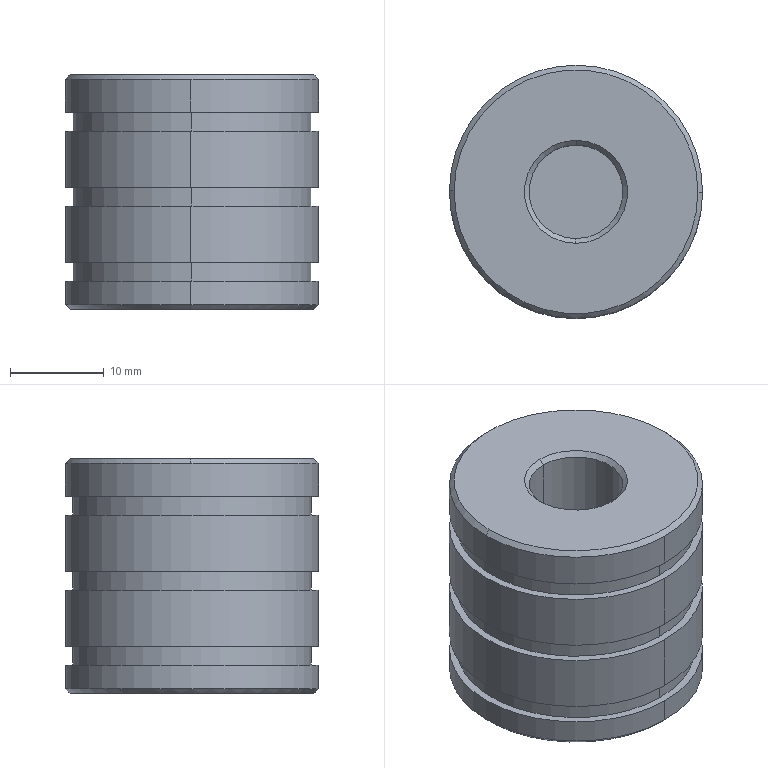Component | SolidWorks | YC1-250-09SecondDropAssembly-1_Coupling-1 | 1 solid | 36 faces | box 27 x 27 x 25 mm | volume 12319 mm3 | cylinder 18 | plane 10 | cone 8 | commonest cylinder face diameters 27 x8 25.4 x6 10 x4 | material Plain Carbon Steel
STEP:
#1=CARTESIAN_POINT('',(0.004281,132.205,-42.775));
#2=VERTEX_POINT('',#1);
#3=CARTESIAN_POINT('',(-0.004281,131.181,-42.775));
#4=VERTEX_POINT('',#3);
#5=CARTESIAN_POINT('',(0.,131.693,-42.775));
#6=DIRECTION('',(0.,0.,1.));
#7=DIRECTION('',(0.008365,1.,0.));
#8=AXIS2_PLACEMENT_3D('',#5,#6,#7);
#9=CIRCLE('',#8,0.5118);
#10=EDGE_CURVE('',#2,#4,#9,.T.);
#11=ORIENTED_EDGE('',*,*,#10,.T.);
#12=CARTESIAN_POINT('',(-0.004446,131.161,-42.755));
#13=VERTEX_POINT('',#12);
#14=CARTESIAN_POINT('',(-0.004446,131.161,-42.755));
#15=DIRECTION('',(-0.005915,-0.7071,0.7071));
#16=VECTOR('',#15,39.37);
#17=LINE('',#14,#16);
#18=EDGE_CURVE('',#4,#13,#17,.T.);
#19=ORIENTED_EDGE('',*,*,#18,.T.);
#20=CARTESIAN_POINT('',(0.004446,132.224,-42.755));
#21=VERTEX_POINT('',#20);
#22=CARTESIAN_POINT('',(0.,131.693,-42.755));
#23=DIRECTION('',(0.,0.,-1.));
#24=DIRECTION('',(0.008365,1.,0.));
#25=AXIS2_PLACEMENT_3D('',#22,#23,#24);
#26=CIRCLE('',#25,0.5315);
#27=EDGE_CURVE('',#13,#21,#26,.T.);
#28=ORIENTED_EDGE('',*,*,#27,.T.);
#29=CARTESIAN_POINT('',(0.004446,132.224,-42.755));
#30=DIRECTION('',(0.005915,0.7071,0.7071));
#31=VECTOR('',#30,39.37);
#32=LINE('',#29,#31);
#33=EDGE_CURVE('',#2,#21,#32,.T.);
#34=ORIENTED_EDGE('',*,*,#33,.F.);
#35=EDGE_LOOP('',(#11,#19,#28,#34));
#36=FACE_OUTER_BOUND('',#35,.T.);
#37=CARTESIAN_POINT('',(0.,131.693,-42.755));
#38=DIRECTION('',(0.,0.,1.));
#39=DIRECTION('',(0.008365,1.,0.));
#40=AXIS2_PLACEMENT_3D('',#37,#38,#39);
#41=CONICAL_SURFACE('',#40,0.5315,0.7854);
#42=ADVANCED_FACE('',(#36),#41,.T.);
#43=CARTESIAN_POINT('',(0.1968,131.691,-42.755));
#44=VERTEX_POINT('',#43);
#45=CARTESIAN_POINT('',(-0.001647,131.496,-42.755));
#46=VERTEX_POINT('',#45);
#47=CARTESIAN_POINT('',(0.,131.693,-42.755));
#48=DIRECTION('',(0.,0.,-1.));
#49=DIRECTION('',(-0.008365,-1.,0.));
#50=AXIS2_PLACEMENT_3D('',#47,#48,#49);
#51=CIRCLE('',#50,0.1969);
#52=EDGE_CURVE('',#44,#46,#51,.T.);
#53=ORIENTED_EDGE('',*,*,#52,.F.);
#54=CARTESIAN_POINT('',(0.2165,131.691,-42.775));
#55=VERTEX_POINT('',#54);
#56=CARTESIAN_POINT('',(0.2165,131.691,-42.775));
#57=DIRECTION('',(0.7071,-0.005915,-0.7071));
#58=VECTOR('',#57,39.37);
#59=LINE('',#56,#58);
#60=EDGE_CURVE('',#44,#55,#59,.T.);
#61=ORIENTED_EDGE('',*,*,#60,.T.);
#62=CARTESIAN_POINT('',(-0.2165,131.695,-42.775));
#63=VERTEX_POINT('',#62);
#64=CARTESIAN_POINT('',(0.,131.693,-42.775));
#65=DIRECTION('',(-0.,0.,-1.));
#66=DIRECTION('',(-1.,0.008365,0.));
#67=AXIS2_PLACEMENT_3D('',#64,#65,#66);
#68=CIRCLE('',#67,0.2165);
#69=EDGE_CURVE('',#55,#63,#68,.T.);
#70=ORIENTED_EDGE('',*,*,#69,.T.);
#71=CARTESIAN_POINT('',(-0.1968,131.695,-42.755));
#72=VERTEX_POINT('',#71);
#73=CARTESIAN_POINT('',(-0.2165,131.695,-42.775));
#74=DIRECTION('',(-0.7071,0.005915,-0.7071));
#75=VECTOR('',#74,39.37);
#76=LINE('',#73,#75);
#77=EDGE_CURVE('',#72,#63,#76,.T.);
#78=ORIENTED_EDGE('',*,*,#77,.F.);
#79=CARTESIAN_POINT('',(0.,131.693,-42.755));
#80=DIRECTION('',(0.,0.,-1.));
#81=DIRECTION('',(-0.008365,-1.,0.));
#82=AXIS2_PLACEMENT_3D('',#79,#80,#81);
#83=CIRCLE('',#82,0.1969);
#84=EDGE_CURVE('',#46,#72,#83,.T.);
#85=ORIENTED_EDGE('',*,*,#84,.F.);
#86=EDGE_LOOP('',(#53,#61,#70,#78,#85));
#87=FACE_OUTER_BOUND('',#86,.T.);
#88=CARTESIAN_POINT('',(0.,131.693,-42.775));
#89=DIRECTION('',(-0.,0.,-1.));
#90=DIRECTION('',(-1.,0.008365,0.));
#91=AXIS2_PLACEMENT_3D('',#88,#89,#90);
#92=CONICAL_SURFACE('',#91,0.2165,0.7854);
#93=ADVANCED_FACE('',(#87),#92,.F.);
#94=ORIENTED_EDGE('',*,*,#27,.F.);
#95=CARTESIAN_POINT('',(-0.004446,131.161,-42.657));
#96=VERTEX_POINT('',#95);
#97=CARTESIAN_POINT('',(-0.004446,131.161,-41.79));
#98=DIRECTION('',(0.,0.,1.));
#99=VECTOR('',#98,39.37);
#100=LINE('',#97,#99);
#101=EDGE_CURVE('',#13,#96,#100,.T.);
#102=ORIENTED_EDGE('',*,*,#101,.T.);
#103=CARTESIAN_POINT('',(0.004446,132.224,-42.657));
#104=VERTEX_POINT('',#103);
#105=CARTESIAN_POINT('',(0.,131.693,-42.657));
#106=DIRECTION('',(0.,0.,-1.));
#107=DIRECTION('',(0.008365,1.,0.));
#108=AXIS2_PLACEMENT_3D('',#105,#106,#107);
#109=CIRCLE('',#108,0.5315);
#110=EDGE_CURVE('',#96,#104,#109,.T.);
#111=ORIENTED_EDGE('',*,*,#110,.T.);
#112=CARTESIAN_POINT('',(0.004446,132.224,-41.79));
#113=DIRECTION('',(0.,0.,1.));
#114=VECTOR('',#113,39.37);
#115=LINE('',#112,#114);
#116=EDGE_CURVE('',#21,#104,#115,.T.);
#117=ORIENTED_EDGE('',*,*,#116,.F.);
#118=EDGE_LOOP('',(#94,#102,#111,#117));
#119=FACE_OUTER_BOUND('',#118,.T.);
#120=CARTESIAN_POINT('',(0.,131.693,-41.79));
#121=DIRECTION('',(0.,0.,1.));
#122=DIRECTION('',(0.008365,1.,0.));
#123=AXIS2_PLACEMENT_3D('',#120,#121,#122);
#124=CYLINDRICAL_SURFACE('',#123,0.5315);
#125=ADVANCED_FACE('',(#119),#124,.T.);
#126=CARTESIAN_POINT('',(0.001647,131.89,-42.755));
#127=VERTEX_POINT('',#126);
#128=CARTESIAN_POINT('',(0.,131.693,-42.755));
#129=DIRECTION('',(0.,0.,-1.));
#130=DIRECTION('',(-0.008365,-1.,0.));
#131=AXIS2_PLACEMENT_3D('',#128,#129,#130);
#132=CIRCLE('',#131,0.1969);
#133=EDGE_CURVE('',#127,#44,#132,.T.);
#134=ORIENTED_EDGE('',*,*,#133,.T.);
#135=ORIENTED_EDGE('',*,*,#52,.T.);
#136=CARTESIAN_POINT('',(-0.001647,131.496,-42.381));
#137=VERTEX_POINT('',#136);
#138=CARTESIAN_POINT('',(-0.001647,131.496,-41.79));
#139=DIRECTION('',(0.,0.,1.));
#140=VECTOR('',#139,39.37);
#141=LINE('',#138,#140);
#142=EDGE_CURVE('',#46,#137,#141,.T.);
#143=ORIENTED_EDGE('',*,*,#142,.T.);
#144=CARTESIAN_POINT('',(0.001647,131.89,-42.381));
#145=VERTEX_POINT('',#144);
#146=CARTESIAN_POINT('',(0.,131.693,-42.381));
#147=DIRECTION('',(0.,0.,-1.));
#148=DIRECTION('',(0.008365,1.,0.));
#149=AXIS2_PLACEMENT_3D('',#146,#147,#148);
#150=CIRCLE('',#149,0.1969);
#151=EDGE_CURVE('',#145,#137,#150,.T.);
#152=ORIENTED_EDGE('',*,*,#151,.F.);
#153=CARTESIAN_POINT('',(0.001647,131.89,-41.79));
#154=DIRECTION('',(0.,0.,1.));
#155=VECTOR('',#154,39.37);
#156=LINE('',#153,#155);
#157=EDGE_CURVE('',#127,#145,#156,.T.);
#158=ORIENTED_EDGE('',*,*,#157,.F.);
#159=EDGE_LOOP('',(#134,#135,#143,#152,#158));
#160=FACE_OUTER_BOUND('',#159,.T.);
#161=CARTESIAN_POINT('',(0.,131.693,-41.79));
#162=DIRECTION('',(0.,0.,1.));
#163=DIRECTION('',(0.008365,1.,0.));
#164=AXIS2_PLACEMENT_3D('',#161,#162,#163);
#165=CYLINDRICAL_SURFACE('',#164,0.1969);
#166=ADVANCED_FACE('',(#160),#165,.F.);
#167=CARTESIAN_POINT('',(-0.004183,131.193,-42.578));
#168=VERTEX_POINT('',#167);
#169=CARTESIAN_POINT('',(0.004183,132.193,-42.578));
#170=VERTEX_POINT('',#169);
#171=CARTESIAN_POINT('',(0.,131.693,-42.578));
#172=DIRECTION('',(0.,0.,-1.));
#173=DIRECTION('',(-0.008365,-1.,0.));
#174=AXIS2_PLACEMENT_3D('',#171,#172,#173);
#175=CIRCLE('',#174,0.5);
#176=EDGE_CURVE('',#168,#170,#175,.T.);
#177=ORIENTED_EDGE('',*,*,#176,.T.);
#178=CARTESIAN_POINT('',(0.004183,132.193,-42.657));
#179=VERTEX_POINT('',#178);
#180=CARTESIAN_POINT('',(0.004183,132.193,-42.578));
#181=DIRECTION('',(0.,0.,-1.));
#182=VECTOR('',#181,39.37);
#183=LINE('',#180,#182);
#184=EDGE_CURVE('',#170,#179,#183,.T.);
#185=ORIENTED_EDGE('',*,*,#184,.T.);
#186=CARTESIAN_POINT('',(-0.004183,131.193,-42.657));
#187=VERTEX_POINT('',#186);
#188=CARTESIAN_POINT('',(0.,131.693,-42.657));
#189=DIRECTION('',(0.,0.,1.));
#190=DIRECTION('',(-0.008365,-1.,0.));
#191=AXIS2_PLACEMENT_3D('',#188,#189,#190);
#192=CIRCLE('',#191,0.5);
#193=EDGE_CURVE('',#179,#187,#192,.T.);
#194=ORIENTED_EDGE('',*,*,#193,.T.);
#195=CARTESIAN_POINT('',(-0.004183,131.193,-42.578));
#196=DIRECTION('',(0.,0.,-1.));
#197=VECTOR('',#196,39.37);
#198=LINE('',#195,#197);
#199=EDGE_CURVE('',#168,#187,#198,.T.);
#200=ORIENTED_EDGE('',*,*,#199,.F.);
#201=EDGE_LOOP('',(#177,#185,#194,#200));
#202=FACE_OUTER_BOUND('',#201,.T.);
#203=CARTESIAN_POINT('',(0.,131.693,-42.578));
#204=DIRECTION('',(0.,0.,-1.));
#205=DIRECTION('',(-0.008365,-1.,0.));
#206=AXIS2_PLACEMENT_3D('',#203,#204,#205);
#207=CYLINDRICAL_SURFACE('',#206,0.5);
#208=ADVANCED_FACE('',(#202),#207,.T.);
#209=CARTESIAN_POINT('',(0.004446,132.224,-42.578));
#210=VERTEX_POINT('',#209);
#211=CARTESIAN_POINT('',(-0.004446,131.161,-42.578));
#212=VERTEX_POINT('',#211);
#213=CARTESIAN_POINT('',(0.,131.693,-42.578));
#214=DIRECTION('',(0.,0.,1.));
#215=DIRECTION('',(0.008365,1.,0.));
#216=AXIS2_PLACEMENT_3D('',#213,#214,#215);
#217=CIRCLE('',#216,0.5315);
#218=EDGE_CURVE('',#210,#212,#217,.T.);
#219=ORIENTED_EDGE('',*,*,#218,.T.);
#220=CARTESIAN_POINT('',(-0.004446,131.161,-42.342));
#221=VERTEX_POINT('',#220);
#222=CARTESIAN_POINT('',(-0.004446,131.161,-41.79));
#223=DIRECTION('',(0.,0.,1.));
#224=VECTOR('',#223,39.37);
#225=LINE('',#222,#224);
#226=EDGE_CURVE('',#212,#221,#225,.T.);
#227=ORIENTED_EDGE('',*,*,#226,.T.);
#228=CARTESIAN_POINT('',(0.004446,132.224,-42.342));
#229=VERTEX_POINT('',#228);
#230=CARTESIAN_POINT('',(0.,131.693,-42.342));
#231=DIRECTION('',(0.,0.,-1.));
#232=DIRECTION('',(0.008365,1.,0.));
#233=AXIS2_PLACEMENT_3D('',#230,#231,#232);
#234=CIRCLE('',#233,0.5315);
#235=EDGE_CURVE('',#221,#229,#234,.T.);
#236=ORIENTED_EDGE('',*,*,#235,.T.);
#237=CARTESIAN_POINT('',(0.004446,132.224,-41.79));
#238=DIRECTION('',(0.,0.,1.));
#239=VECTOR('',#238,39.37);
#240=LINE('',#237,#239);
#241=EDGE_CURVE('',#210,#229,#240,.T.);
#242=ORIENTED_EDGE('',*,*,#241,.F.);
#243=EDGE_LOOP('',(#219,#227,#236,#242));
#244=FACE_OUTER_BOUND('',#243,.T.);
#245=CARTESIAN_POINT('',(0.,131.693,-41.79));
#246=DIRECTION('',(0.,0.,1.));
#247=DIRECTION('',(0.008365,1.,0.));
#248=AXIS2_PLACEMENT_3D('',#245,#246,#247);
#249=CYLINDRICAL_SURFACE('',#248,0.5315);
#250=ADVANCED_FACE('',(#244),#249,.T.);
#251=CARTESIAN_POINT('',(-0.004183,131.193,-42.263));
#252=VERTEX_POINT('',#251);
#253=CARTESIAN_POINT('',(0.004183,132.193,-42.263));
#254=VERTEX_POINT('',#253);
#255=CARTESIAN_POINT('',(0.,131.693,-42.263));
#256=DIRECTION('',(0.,0.,-1.));
#257=DIRECTION('',(-0.008365,-1.,0.));
#258=AXIS2_PLACEMENT_3D('',#255,#256,#257);
#259=CIRCLE('',#258,0.5);
#260=EDGE_CURVE('',#252,#254,#259,.T.);
#261=ORIENTED_EDGE('',*,*,#260,.T.);
#262=CARTESIAN_POINT('',(0.004183,132.193,-42.342));
#263=VERTEX_POINT('',#262);
#264=CARTESIAN_POINT('',(0.004183,132.193,-42.263));
#265=DIRECTION('',(0.,0.,-1.));
#266=VECTOR('',#265,39.37);
#267=LINE('',#264,#266);
#268=EDGE_CURVE('',#254,#263,#267,.T.);
#269=ORIENTED_EDGE('',*,*,#268,.T.);
#270=CARTESIAN_POINT('',(-0.004183,131.193,-42.342));
#271=VERTEX_POINT('',#270);
#272=CARTESIAN_POINT('',(0.,131.693,-42.342));
#273=DIRECTION('',(0.,0.,1.));
#274=DIRECTION('',(-0.008365,-1.,0.));
#275=AXIS2_PLACEMENT_3D('',#272,#273,#274);
#276=CIRCLE('',#275,0.5);
#277=EDGE_CURVE('',#263,#271,#276,.T.);
#278=ORIENTED_EDGE('',*,*,#277,.T.);
#279=CARTESIAN_POINT('',(-0.004183,131.193,-42.263));
#280=DIRECTION('',(0.,0.,-1.));
#281=VECTOR('',#280,39.37);
#282=LINE('',#279,#281);
#283=EDGE_CURVE('',#252,#271,#282,.T.);
#284=ORIENTED_EDGE('',*,*,#283,.F.);
#285=EDGE_LOOP('',(#261,#269,#278,#284));
#286=FACE_OUTER_BOUND('',#285,.T.);
#287=CARTESIAN_POINT('',(0.,131.693,-42.263));
#288=DIRECTION('',(0.,0.,-1.));
#289=DIRECTION('',(-0.008365,-1.,0.));
#290=AXIS2_PLACEMENT_3D('',#287,#288,#289);
#291=CYLINDRICAL_SURFACE('',#290,0.5);
#292=ADVANCED_FACE('',(#286),#291,.T.);
#293=CARTESIAN_POINT('',(0.004446,132.224,-42.263));
#294=VERTEX_POINT('',#293);
#295=CARTESIAN_POINT('',(-0.004446,131.161,-42.263));
#296=VERTEX_POINT('',#295);
#297=CARTESIAN_POINT('',(0.,131.693,-42.263));
#298=DIRECTION('',(0.,0.,1.));
#299=DIRECTION('',(0.008365,1.,0.));
#300=AXIS2_PLACEMENT_3D('',#297,#298,#299);
#301=CIRCLE('',#300,0.5315);
#302=EDGE_CURVE('',#294,#296,#301,.T.);
#303=ORIENTED_EDGE('',*,*,#302,.T.);
#304=CARTESIAN_POINT('',(-0.004446,131.161,-42.027));
#305=VERTEX_POINT('',#304);
#306=CARTESIAN_POINT('',(-0.004446,131.161,-41.79));
#307=DIRECTION('',(0.,0.,1.));
#308=VECTOR('',#307,39.37);
#309=LINE('',#306,#308);
#310=EDGE_CURVE('',#296,#305,#309,.T.);
#311=ORIENTED_EDGE('',*,*,#310,.T.);
#312=CARTESIAN_POINT('',(0.004446,132.224,-42.027));
#313=VERTEX_POINT('',#312);
#314=CARTESIAN_POINT('',(0.,131.693,-42.027));
#315=DIRECTION('',(0.,0.,-1.));
#316=DIRECTION('',(0.008365,1.,0.));
#317=AXIS2_PLACEMENT_3D('',#314,#315,#316);
#318=CIRCLE('',#317,0.5315);
#319=EDGE_CURVE('',#305,#313,#318,.T.);
#320=ORIENTED_EDGE('',*,*,#319,.T.);
#321=CARTESIAN_POINT('',(0.004446,132.224,-41.79));
#322=DIRECTION('',(0.,0.,1.));
#323=VECTOR('',#322,39.37);
#324=LINE('',#321,#323);
#325=EDGE_CURVE('',#294,#313,#324,.T.);
#326=ORIENTED_EDGE('',*,*,#325,.F.);
#327=EDGE_LOOP('',(#303,#311,#320,#326));
#328=FACE_OUTER_BOUND('',#327,.T.);
#329=CARTESIAN_POINT('',(0.,131.693,-41.79));
#330=DIRECTION('',(0.,0.,1.));
#331=DIRECTION('',(0.008365,1.,0.));
#332=AXIS2_PLACEMENT_3D('',#329,#330,#331);
#333=CYLINDRICAL_SURFACE('',#332,0.5315);
#334=ADVANCED_FACE('',(#328),#333,.T.);
#335=CARTESIAN_POINT('',(-0.004183,131.193,-41.948));
#336=VERTEX_POINT('',#335);
#337=CARTESIAN_POINT('',(0.004183,132.193,-41.948));
#338=VERTEX_POINT('',#337);
#339=CARTESIAN_POINT('',(0.,131.693,-41.948));
#340=DIRECTION('',(0.,0.,-1.));
#341=DIRECTION('',(-0.008365,-1.,0.));
#342=AXIS2_PLACEMENT_3D('',#339,#340,#341);
#343=CIRCLE('',#342,0.5);
#344=EDGE_CURVE('',#336,#338,#343,.T.);
#345=ORIENTED_EDGE('',*,*,#344,.T.);
#346=CARTESIAN_POINT('',(0.004183,132.193,-42.027));
#347=VERTEX_POINT('',#346);
#348=CARTESIAN_POINT('',(0.004183,132.193,-42.755));
#349=DIRECTION('',(0.,0.,-1.));
#350=VECTOR('',#349,39.37);
#351=LINE('',#348,#350);
#352=EDGE_CURVE('',#338,#347,#351,.T.);
#353=ORIENTED_EDGE('',*,*,#352,.T.);
#354=CARTESIAN_POINT('',(-0.004183,131.193,-42.027));
#355=VERTEX_POINT('',#354);
#356=CARTESIAN_POINT('',(0.,131.693,-42.027));
#357=DIRECTION('',(0.,0.,1.));
#358=DIRECTION('',(-0.008365,-1.,0.));
#359=AXIS2_PLACEMENT_3D('',#356,#357,#358);
#360=CIRCLE('',#359,0.5);
#361=EDGE_CURVE('',#347,#355,#360,.T.);
#362=ORIENTED_EDGE('',*,*,#361,.T.);
#363=CARTESIAN_POINT('',(-0.004183,131.193,-42.755));
#364=DIRECTION('',(0.,0.,-1.));
#365=VECTOR('',#364,39.37);
#366=LINE('',#363,#365);
#367=EDGE_CURVE('',#336,#355,#366,.T.);
#368=ORIENTED_EDGE('',*,*,#367,.F.);
#369=EDGE_LOOP('',(#345,#353,#362,#368));
#370=FACE_OUTER_BOUND('',#369,.T.);
#371=CARTESIAN_POINT('',(0.,131.693,-42.755));
#372=DIRECTION('',(0.,0.,-1.));
#373=DIRECTION('',(-0.008365,-1.,0.));
#374=AXIS2_PLACEMENT_3D('',#371,#372,#373);
#375=CYLINDRICAL_SURFACE('',#374,0.5);
#376=ADVANCED_FACE('',(#370),#375,.T.);
#377=CARTESIAN_POINT('',(0.004446,132.224,-41.948));
#378=VERTEX_POINT('',#377);
#379=CARTESIAN_POINT('',(-0.004446,131.161,-41.948));
#380=VERTEX_POINT('',#379);
#381=CARTESIAN_POINT('',(0.,131.693,-41.948));
#382=DIRECTION('',(0.,0.,1.));
#383=DIRECTION('',(0.008365,1.,0.));
#384=AXIS2_PLACEMENT_3D('',#381,#382,#383);
#385=CIRCLE('',#384,0.5315);
#386=EDGE_CURVE('',#378,#380,#385,.T.);
#387=ORIENTED_EDGE('',*,*,#386,.T.);
#388=CARTESIAN_POINT('',(-0.004446,131.161,-41.81));
#389=VERTEX_POINT('',#388);
#390=CARTESIAN_POINT('',(-0.004446,131.161,-41.79));
#391=DIRECTION('',(0.,0.,1.));
#392=VECTOR('',#391,39.37);
#393=LINE('',#390,#392);
#394=EDGE_CURVE('',#380,#389,#393,.T.);
#395=ORIENTED_EDGE('',*,*,#394,.T.);
#396=CARTESIAN_POINT('',(-0.5315,131.697,-41.81));
#397=VERTEX_POINT('',#396);
#398=CARTESIAN_POINT('',(0.,131.693,-41.81));
#399=DIRECTION('',(0.,0.,-1.));
#400=DIRECTION('',(0.008365,1.,0.));
#401=AXIS2_PLACEMENT_3D('',#398,#399,#400);
#402=CIRCLE('',#401,0.5315);
#403=EDGE_CURVE('',#389,#397,#402,.T.);
#404=ORIENTED_EDGE('',*,*,#403,.T.);
#405=CARTESIAN_POINT('',(0.004446,132.224,-41.81));
#406=VERTEX_POINT('',#405);
#407=CARTESIAN_POINT('',(0.,131.693,-41.81));
#408=DIRECTION('',(0.,0.,-1.));
#409=DIRECTION('',(0.008365,1.,0.));
#410=AXIS2_PLACEMENT_3D('',#407,#408,#409);
#411=CIRCLE('',#410,0.5315);
#412=EDGE_CURVE('',#397,#406,#411,.T.);
#413=ORIENTED_EDGE('',*,*,#412,.T.);
#414=CARTESIAN_POINT('',(0.004446,132.224,-41.79));
#415=DIRECTION('',(0.,0.,1.));
#416=VECTOR('',#415,39.37);
#417=LINE('',#414,#416);
#418=EDGE_CURVE('',#378,#406,#417,.T.);
#419=ORIENTED_EDGE('',*,*,#418,.F.);
#420=EDGE_LOOP('',(#387,#395,#404,#413,#419));
#421=FACE_OUTER_BOUND('',#420,.T.);
#422=CARTESIAN_POINT('',(0.,131.693,-41.79));
#423=DIRECTION('',(0.,0.,1.));
#424=DIRECTION('',(0.008365,1.,0.));
#425=AXIS2_PLACEMENT_3D('',#422,#423,#424);
#426=CYLINDRICAL_SURFACE('',#425,0.5315);
#427=ADVANCED_FACE('',(#421),#426,.T.);
#428=CARTESIAN_POINT('',(-0.5118,131.697,-41.79));
#429=VERTEX_POINT('',#428);
#430=CARTESIAN_POINT('',(0.5118,131.689,-41.79));
#431=VERTEX_POINT('',#430);
#432=CARTESIAN_POINT('',(0.,131.693,-41.79));
#433=DIRECTION('',(-0.,0.,-1.));
#434=DIRECTION('',(-1.,0.008365,0.));
#435=AXIS2_PLACEMENT_3D('',#432,#433,#434);
#436=CIRCLE('',#435,0.5118);
#437=EDGE_CURVE('',#429,#431,#436,.T.);
#438=ORIENTED_EDGE('',*,*,#437,.T.);
#439=CARTESIAN_POINT('',(0.5315,131.688,-41.81));
#440=VERTEX_POINT('',#439);
#441=CARTESIAN_POINT('',(0.5315,131.688,-41.81));
#442=DIRECTION('',(0.7071,-0.005915,-0.7071));
#443=VECTOR('',#442,39.37);
#444=LINE('',#441,#443);
#445=EDGE_CURVE('',#431,#440,#444,.T.);
#446=ORIENTED_EDGE('',*,*,#445,.T.);
#447=CARTESIAN_POINT('',(0.,131.693,-41.81));
#448=DIRECTION('',(0.,0.,-1.));
#449=DIRECTION('',(0.008365,1.,0.));
#450=AXIS2_PLACEMENT_3D('',#447,#448,#449);
#451=CIRCLE('',#450,0.5315);
#452=EDGE_CURVE('',#406,#440,#451,.T.);
#453=ORIENTED_EDGE('',*,*,#452,.F.);
#454=ORIENTED_EDGE('',*,*,#412,.F.);
#455=CARTESIAN_POINT('',(-0.5315,131.697,-41.81));
#456=DIRECTION('',(-0.7071,0.005915,-0.7071));
#457=VECTOR('',#456,39.37);
#458=LINE('',#455,#457);
#459=EDGE_CURVE('',#429,#397,#458,.T.);
#460=ORIENTED_EDGE('',*,*,#459,.F.);
#461=EDGE_LOOP('',(#438,#446,#453,#454,#460));
#462=FACE_OUTER_BOUND('',#461,.T.);
#463=CARTESIAN_POINT('',(0.,131.693,-41.81));
#464=DIRECTION('',(-0.,0.,-1.));
#465=DIRECTION('',(-1.,0.008365,0.));
#466=AXIS2_PLACEMENT_3D('',#463,#464,#465);
#467=CONICAL_SURFACE('',#466,0.5315,0.7854);
#468=ADVANCED_FACE('',(#462),#467,.T.);
#469=CARTESIAN_POINT('',(-0.001647,131.496,-41.81));
#470=VERTEX_POINT('',#469);
#471=CARTESIAN_POINT('',(0.001647,131.89,-41.81));
#472=VERTEX_POINT('',#471);
#473=CARTESIAN_POINT('',(0.,131.693,-41.81));
#474=DIRECTION('',(0.,0.,1.));
#475=DIRECTION('',(0.008365,1.,0.));
#476=AXIS2_PLACEMENT_3D('',#473,#474,#475);
#477=CIRCLE('',#476,0.1969);
#478=EDGE_CURVE('',#470,#472,#477,.T.);
#479=ORIENTED_EDGE('',*,*,#478,.F.);
#480=CARTESIAN_POINT('',(-0.001811,131.476,-41.79));
#481=VERTEX_POINT('',#480);
#482=CARTESIAN_POINT('',(-0.001811,131.476,-41.79));
#483=DIRECTION('',(-0.005915,-0.7071,0.7071));
#484=VECTOR('',#483,39.37);
#485=LINE('',#482,#484);
#486=EDGE_CURVE('',#470,#481,#485,.T.);
#487=ORIENTED_EDGE('',*,*,#486,.T.);
#488=CARTESIAN_POINT('',(0.001811,131.909,-41.79));
#489=VERTEX_POINT('',#488);
#490=CARTESIAN_POINT('',(0.,131.693,-41.79));
#491=DIRECTION('',(0.,0.,1.));
#492=DIRECTION('',(0.008365,1.,0.));
#493=AXIS2_PLACEMENT_3D('',#490,#491,#492);
#494=CIRCLE('',#493,0.2165);
#495=EDGE_CURVE('',#481,#489,#494,.T.);
#496=ORIENTED_EDGE('',*,*,#495,.T.);
#497=CARTESIAN_POINT('',(0.001811,131.909,-41.79));
#498=DIRECTION('',(0.005915,0.7071,0.7071));
#499=VECTOR('',#498,39.37);
#500=LINE('',#497,#499);
#501=EDGE_CURVE('',#472,#489,#500,.T.);
#502=ORIENTED_EDGE('',*,*,#501,.F.);
#503=EDGE_LOOP('',(#479,#487,#496,#502));
#504=FACE_OUTER_BOUND('',#503,.T.);
#505=CARTESIAN_POINT('',(0.,131.693,-41.79));
#506=DIRECTION('',(0.,0.,1.));
#507=DIRECTION('',(0.008365,1.,0.));
#508=AXIS2_PLACEMENT_3D('',#505,#506,#507);
#509=CONICAL_SURFACE('',#508,0.2165,0.7854);
#510=ADVANCED_FACE('',(#504),#509,.F.);
#511=CARTESIAN_POINT('',(-0.001647,131.496,-42.184));
#512=VERTEX_POINT('',#511);
#513=CARTESIAN_POINT('',(0.001647,131.89,-42.184));
#514=VERTEX_POINT('',#513);
#515=CARTESIAN_POINT('',(0.,131.693,-42.184));
#516=DIRECTION('',(0.,0.,1.));
#517=DIRECTION('',(0.008365,1.,0.));
#518=AXIS2_PLACEMENT_3D('',#515,#516,#517);
#519=CIRCLE('',#518,0.1969);
#520=EDGE_CURVE('',#512,#514,#519,.T.);
#521=ORIENTED_EDGE('',*,*,#520,.F.);
#522=CARTESIAN_POINT('',(-0.001647,131.496,-41.79));
#523=DIRECTION('',(0.,0.,1.));
#524=VECTOR('',#523,39.37);
#525=LINE('',#522,#524);
#526=EDGE_CURVE('',#512,#470,#525,.T.);
#527=ORIENTED_EDGE('',*,*,#526,.T.);
#528=ORIENTED_EDGE('',*,*,#478,.T.);
#529=CARTESIAN_POINT('',(0.001647,131.89,-41.79));
#530=DIRECTION('',(0.,0.,1.));
#531=VECTOR('',#530,39.37);
#532=LINE('',#529,#531);
#533=EDGE_CURVE('',#514,#472,#532,.T.);
#534=ORIENTED_EDGE('',*,*,#533,.F.);
#535=EDGE_LOOP('',(#521,#527,#528,#534));
#536=FACE_OUTER_BOUND('',#535,.T.);
#537=CARTESIAN_POINT('',(0.,131.693,-41.79));
#538=DIRECTION('',(0.,0.,1.));
#539=DIRECTION('',(0.008365,1.,0.));
#540=AXIS2_PLACEMENT_3D('',#537,#538,#539);
#541=CYLINDRICAL_SURFACE('',#540,0.1969);
#542=ADVANCED_FACE('',(#536),#541,.F.);
#543=ORIENTED_EDGE('',*,*,#10,.F.);
#544=CARTESIAN_POINT('',(0.,131.693,-42.775));
#545=DIRECTION('',(0.,0.,1.));
#546=DIRECTION('',(0.008365,1.,0.));
#547=AXIS2_PLACEMENT_3D('',#544,#545,#546);
#548=CIRCLE('',#547,0.5118);
#549=EDGE_CURVE('',#4,#2,#548,.T.);
#550=ORIENTED_EDGE('',*,*,#549,.F.);
#551=EDGE_LOOP('',(#543,#550));
#552=FACE_OUTER_BOUND('',#551,.T.);
#553=CARTESIAN_POINT('',(0.,131.693,-42.775));
#554=DIRECTION('',(-0.,0.,-1.));
#555=DIRECTION('',(-1.,0.008365,0.));
#556=AXIS2_PLACEMENT_3D('',#553,#554,#555);
#557=CIRCLE('',#556,0.2165);
#558=EDGE_CURVE('',#63,#55,#557,.T.);
#559=ORIENTED_EDGE('',*,*,#558,.F.);
#560=ORIENTED_EDGE('',*,*,#69,.F.);
#561=EDGE_LOOP('',(#559,#560));
#562=FACE_BOUND('',#561,.T.);
#563=CARTESIAN_POINT('',(-0.1968,131.695,-42.775));
#564=DIRECTION('',(0.,0.,1.));
#565=DIRECTION('',(0.008365,1.,0.));
#566=AXIS2_PLACEMENT_3D('',#563,#564,#565);
#567=PLANE('',#566);
#568=ADVANCED_FACE('',(#552,#562),#567,.F.);
#569=ORIENTED_EDGE('',*,*,#18,.F.);
#570=ORIENTED_EDGE('',*,*,#549,.T.);
#571=ORIENTED_EDGE('',*,*,#33,.T.);
#572=CARTESIAN_POINT('',(0.,131.693,-42.755));
#573=DIRECTION('',(0.,0.,-1.));
#574=DIRECTION('',(0.008365,1.,0.));
#575=AXIS2_PLACEMENT_3D('',#572,#573,#574);
#576=CIRCLE('',#575,0.5315);
#577=EDGE_CURVE('',#21,#13,#576,.T.);
#578=ORIENTED_EDGE('',*,*,#577,.T.);
#579=EDGE_LOOP('',(#569,#570,#571,#578));
#580=FACE_OUTER_BOUND('',#579,.T.);
#581=CARTESIAN_POINT('',(0.,131.693,-42.755));
#582=DIRECTION('',(0.,0.,1.));
#583=DIRECTION('',(0.008365,1.,0.));
#584=AXIS2_PLACEMENT_3D('',#581,#582,#583);
#585=CONICAL_SURFACE('',#584,0.5315,0.7854);
#586=ADVANCED_FACE('',(#580),#585,.T.);
#587=ORIENTED_EDGE('',*,*,#60,.F.);
#588=ORIENTED_EDGE('',*,*,#133,.F.);
#589=CARTESIAN_POINT('',(0.,131.693,-42.755));
#590=DIRECTION('',(0.,0.,-1.));
#591=DIRECTION('',(-0.008365,-1.,0.));
#592=AXIS2_PLACEMENT_3D('',#589,#590,#591);
#593=CIRCLE('',#592,0.1969);
#594=EDGE_CURVE('',#72,#127,#593,.T.);
#595=ORIENTED_EDGE('',*,*,#594,.F.);
#596=ORIENTED_EDGE('',*,*,#77,.T.);
#597=ORIENTED_EDGE('',*,*,#558,.T.);
#598=EDGE_LOOP('',(#587,#588,#595,#596,#597));
#599=FACE_OUTER_BOUND('',#598,.T.);
#600=CARTESIAN_POINT('',(0.,131.693,-42.775));
#601=DIRECTION('',(-0.,0.,-1.));
#602=DIRECTION('',(-1.,0.008365,0.));
#603=AXIS2_PLACEMENT_3D('',#600,#601,#602);
#604=CONICAL_SURFACE('',#603,0.2165,0.7854);
#605=ADVANCED_FACE('',(#599),#604,.F.);
#606=ORIENTED_EDGE('',*,*,#101,.F.);
#607=ORIENTED_EDGE('',*,*,#577,.F.);
#608=ORIENTED_EDGE('',*,*,#116,.T.);
#609=CARTESIAN_POINT('',(0.,131.693,-42.657));
#610=DIRECTION('',(0.,0.,-1.));
#611=DIRECTION('',(0.008365,1.,0.));
#612=AXIS2_PLACEMENT_3D('',#609,#610,#611);
#613=CIRCLE('',#612,0.5315);
#614=EDGE_CURVE('',#104,#96,#613,.T.);
#615=ORIENTED_EDGE('',*,*,#614,.T.);
#616=EDGE_LOOP('',(#606,#607,#608,#615));
#617=FACE_OUTER_BOUND('',#616,.T.);
#618=CARTESIAN_POINT('',(0.,131.693,-41.79));
#619=DIRECTION('',(0.,0.,1.));
#620=DIRECTION('',(0.008365,1.,0.));
#621=AXIS2_PLACEMENT_3D('',#618,#619,#620);
#622=CYLINDRICAL_SURFACE('',#621,0.5315);
#623=ADVANCED_FACE('',(#617),#622,.T.);
#624=ORIENTED_EDGE('',*,*,#142,.F.);
#625=ORIENTED_EDGE('',*,*,#84,.T.);
#626=ORIENTED_EDGE('',*,*,#594,.T.);
#627=ORIENTED_EDGE('',*,*,#157,.T.);
#628=CARTESIAN_POINT('',(0.,131.693,-42.381));
#629=DIRECTION('',(0.,0.,-1.));
#630=DIRECTION('',(0.008365,1.,0.));
#631=AXIS2_PLACEMENT_3D('',#628,#629,#630);
#632=CIRCLE('',#631,0.1969);
#633=EDGE_CURVE('',#137,#145,#632,.T.);
#634=ORIENTED_EDGE('',*,*,#633,.F.);
#635=EDGE_LOOP('',(#624,#625,#626,#627,#634));
#636=FACE_OUTER_BOUND('',#635,.T.);
#637=CARTESIAN_POINT('',(0.,131.693,-41.79));
#638=DIRECTION('',(0.,0.,1.));
#639=DIRECTION('',(0.008365,1.,0.));
#640=AXIS2_PLACEMENT_3D('',#637,#638,#639);
#641=CYLINDRICAL_SURFACE('',#640,0.1969);
#642=ADVANCED_FACE('',(#636),#641,.F.);
#643=CARTESIAN_POINT('',(0.,131.693,-42.657));
#644=DIRECTION('',(0.,0.,1.));
#645=DIRECTION('',(-0.008365,-1.,0.));
#646=AXIS2_PLACEMENT_3D('',#643,#644,#645);
#647=CIRCLE('',#646,0.5);
#648=EDGE_CURVE('',#187,#179,#647,.T.);
#649=ORIENTED_EDGE('',*,*,#648,.F.);
#650=ORIENTED_EDGE('',*,*,#193,.F.);
#651=EDGE_LOOP('',(#649,#650));
#652=FACE_BOUND('',#651,.T.);
#653=ORIENTED_EDGE('',*,*,#614,.F.);
#654=ORIENTED_EDGE('',*,*,#110,.F.);
#655=EDGE_LOOP('',(#653,#654));
#656=FACE_OUTER_BOUND('',#655,.T.);
#657=CARTESIAN_POINT('',(-0.5,131.697,-42.657));
#658=DIRECTION('',(0.,0.,-1.));
#659=DIRECTION('',(-0.008365,-1.,0.));
#660=AXIS2_PLACEMENT_3D('',#657,#658,#659);
#661=PLANE('',#660);
#662=ADVANCED_FACE('',(#652,#656),#661,.F.);
#663=ORIENTED_EDGE('',*,*,#151,.T.);
#664=ORIENTED_EDGE('',*,*,#633,.T.);
#665=EDGE_LOOP('',(#663,#664));
#666=FACE_OUTER_BOUND('',#665,.T.);
#667=CARTESIAN_POINT('',(0.,131.693,-42.381));
#668=DIRECTION('',(0.,0.,1.));
#669=DIRECTION('',(0.008365,1.,0.));
#670=AXIS2_PLACEMENT_3D('',#667,#668,#669);
#671=PLANE('',#670);
#672=ADVANCED_FACE('',(#666),#671,.F.);
#673=ORIENTED_EDGE('',*,*,#184,.F.);
#674=CARTESIAN_POINT('',(0.,131.693,-42.578));
#675=DIRECTION('',(0.,0.,-1.));
#676=DIRECTION('',(-0.008365,-1.,0.));
#677=AXIS2_PLACEMENT_3D('',#674,#675,#676);
#678=CIRCLE('',#677,0.5);
#679=EDGE_CURVE('',#170,#168,#678,.T.);
#680=ORIENTED_EDGE('',*,*,#679,.T.);
#681=ORIENTED_EDGE('',*,*,#199,.T.);
#682=ORIENTED_EDGE('',*,*,#648,.T.);
#683=EDGE_LOOP('',(#673,#680,#681,#682));
#684=FACE_OUTER_BOUND('',#683,.T.);
#685=CARTESIAN_POINT('',(0.,131.693,-42.578));
#686=DIRECTION('',(0.,0.,-1.));
#687=DIRECTION('',(-0.008365,-1.,0.));
#688=AXIS2_PLACEMENT_3D('',#685,#686,#687);
#689=CYLINDRICAL_SURFACE('',#688,0.5);
#690=ADVANCED_FACE('',(#684),#689,.T.);
#691=ORIENTED_EDGE('',*,*,#218,.F.);
#692=CARTESIAN_POINT('',(0.,131.693,-42.578));
#693=DIRECTION('',(0.,0.,1.));
#694=DIRECTION('',(0.008365,1.,0.));
#695=AXIS2_PLACEMENT_3D('',#692,#693,#694);
#696=CIRCLE('',#695,0.5315);
#697=EDGE_CURVE('',#212,#210,#696,.T.);
#698=ORIENTED_EDGE('',*,*,#697,.F.);
#699=EDGE_LOOP('',(#691,#698));
#700=FACE_OUTER_BOUND('',#699,.T.);
#701=ORIENTED_EDGE('',*,*,#176,.F.);
#702=ORIENTED_EDGE('',*,*,#679,.F.);
#703=EDGE_LOOP('',(#701,#702));
#704=FACE_BOUND('',#703,.T.);
#705=CARTESIAN_POINT('',(-0.5315,131.697,-42.578));
#706=DIRECTION('',(0.,0.,1.));
#707=DIRECTION('',(0.008365,1.,0.));
#708=AXIS2_PLACEMENT_3D('',#705,#706,#707);
#709=PLANE('',#708);
#710=ADVANCED_FACE('',(#700,#704),#709,.F.);
#711=ORIENTED_EDGE('',*,*,#226,.F.);
#712=ORIENTED_EDGE('',*,*,#697,.T.);
#713=ORIENTED_EDGE('',*,*,#241,.T.);
#714=CARTESIAN_POINT('',(0.,131.693,-42.342));
#715=DIRECTION('',(0.,0.,-1.));
#716=DIRECTION('',(0.008365,1.,0.));
#717=AXIS2_PLACEMENT_3D('',#714,#715,#716);
#718=CIRCLE('',#717,0.5315);
#719=EDGE_CURVE('',#229,#221,#718,.T.);
#720=ORIENTED_EDGE('',*,*,#719,.T.);
#721=EDGE_LOOP('',(#711,#712,#713,#720));
#722=FACE_OUTER_BOUND('',#721,.T.);
#723=CARTESIAN_POINT('',(0.,131.693,-41.79));
#724=DIRECTION('',(0.,0.,1.));
#725=DIRECTION('',(0.008365,1.,0.));
#726=AXIS2_PLACEMENT_3D('',#723,#724,#725);
#727=CYLINDRICAL_SURFACE('',#726,0.5315);
#728=ADVANCED_FACE('',(#722),#727,.T.);
#729=CARTESIAN_POINT('',(0.,131.693,-42.342));
#730=DIRECTION('',(0.,0.,1.));
#731=DIRECTION('',(-0.008365,-1.,0.));
#732=AXIS2_PLACEMENT_3D('',#729,#730,#731);
#733=CIRCLE('',#732,0.5);
#734=EDGE_CURVE('',#271,#263,#733,.T.);
#735=ORIENTED_EDGE('',*,*,#734,.F.);
#736=ORIENTED_EDGE('',*,*,#277,.F.);
#737=EDGE_LOOP('',(#735,#736));
#738=FACE_BOUND('',#737,.T.);
#739=ORIENTED_EDGE('',*,*,#719,.F.);
#740=ORIENTED_EDGE('',*,*,#235,.F.);
#741=EDGE_LOOP('',(#739,#740));
#742=FACE_OUTER_BOUND('',#741,.T.);
#743=CARTESIAN_POINT('',(-0.5,131.697,-42.342));
#744=DIRECTION('',(0.,0.,-1.));
#745=DIRECTION('',(-0.008365,-1.,0.));
#746=AXIS2_PLACEMENT_3D('',#743,#744,#745);
#747=PLANE('',#746);
#748=ADVANCED_FACE('',(#738,#742),#747,.F.);
#749=ORIENTED_EDGE('',*,*,#268,.F.);
#750=CARTESIAN_POINT('',(0.,131.693,-42.263));
#751=DIRECTION('',(0.,0.,-1.));
#752=DIRECTION('',(-0.008365,-1.,0.));
#753=AXIS2_PLACEMENT_3D('',#750,#751,#752);
#754=CIRCLE('',#753,0.5);
#755=EDGE_CURVE('',#254,#252,#754,.T.);
#756=ORIENTED_EDGE('',*,*,#755,.T.);
#757=ORIENTED_EDGE('',*,*,#283,.T.);
#758=ORIENTED_EDGE('',*,*,#734,.T.);
#759=EDGE_LOOP('',(#749,#756,#757,#758));
#760=FACE_OUTER_BOUND('',#759,.T.);
#761=CARTESIAN_POINT('',(0.,131.693,-42.263));
#762=DIRECTION('',(0.,0.,-1.));
#763=DIRECTION('',(-0.008365,-1.,0.));
#764=AXIS2_PLACEMENT_3D('',#761,#762,#763);
#765=CYLINDRICAL_SURFACE('',#764,0.5);
#766=ADVANCED_FACE('',(#760),#765,.T.);
#767=ORIENTED_EDGE('',*,*,#302,.F.);
#768=CARTESIAN_POINT('',(0.,131.693,-42.263));
#769=DIRECTION('',(0.,0.,1.));
#770=DIRECTION('',(0.008365,1.,0.));
#771=AXIS2_PLACEMENT_3D('',#768,#769,#770);
#772=CIRCLE('',#771,0.5315);
#773=EDGE_CURVE('',#296,#294,#772,.T.);
#774=ORIENTED_EDGE('',*,*,#773,.F.);
#775=EDGE_LOOP('',(#767,#774));
#776=FACE_OUTER_BOUND('',#775,.T.);
#777=ORIENTED_EDGE('',*,*,#260,.F.);
#778=ORIENTED_EDGE('',*,*,#755,.F.);
#779=EDGE_LOOP('',(#777,#778));
#780=FACE_BOUND('',#779,.T.);
#781=CARTESIAN_POINT('',(-0.5315,131.697,-42.263));
#782=DIRECTION('',(0.,0.,1.));
#783=DIRECTION('',(0.008365,1.,0.));
#784=AXIS2_PLACEMENT_3D('',#781,#782,#783);
#785=PLANE('',#784);
#786=ADVANCED_FACE('',(#776,#780),#785,.F.);
#787=ORIENTED_EDGE('',*,*,#310,.F.);
#788=ORIENTED_EDGE('',*,*,#773,.T.);
#789=ORIENTED_EDGE('',*,*,#325,.T.);
#790=CARTESIAN_POINT('',(0.,131.693,-42.027));
#791=DIRECTION('',(0.,0.,-1.));
#792=DIRECTION('',(0.008365,1.,0.));
#793=AXIS2_PLACEMENT_3D('',#790,#791,#792);
#794=CIRCLE('',#793,0.5315);
#795=EDGE_CURVE('',#313,#305,#794,.T.);
#796=ORIENTED_EDGE('',*,*,#795,.T.);
#797=EDGE_LOOP('',(#787,#788,#789,#796));
#798=FACE_OUTER_BOUND('',#797,.T.);
#799=CARTESIAN_POINT('',(0.,131.693,-41.79));
#800=DIRECTION('',(0.,0.,1.));
#801=DIRECTION('',(0.008365,1.,0.));
#802=AXIS2_PLACEMENT_3D('',#799,#800,#801);
#803=CYLINDRICAL_SURFACE('',#802,0.5315);
#804=ADVANCED_FACE('',(#798),#803,.T.);
#805=CARTESIAN_POINT('',(0.,131.693,-42.027));
#806=DIRECTION('',(0.,0.,1.));
#807=DIRECTION('',(-0.008365,-1.,0.));
#808=AXIS2_PLACEMENT_3D('',#805,#806,#807);
#809=CIRCLE('',#808,0.5);
#810=EDGE_CURVE('',#355,#347,#809,.T.);
#811=ORIENTED_EDGE('',*,*,#810,.F.);
#812=ORIENTED_EDGE('',*,*,#361,.F.);
#813=EDGE_LOOP('',(#811,#812));
#814=FACE_BOUND('',#813,.T.);
#815=ORIENTED_EDGE('',*,*,#795,.F.);
#816=ORIENTED_EDGE('',*,*,#319,.F.);
#817=EDGE_LOOP('',(#815,#816));
#818=FACE_OUTER_BOUND('',#817,.T.);
#819=CARTESIAN_POINT('',(-0.5,131.697,-42.027));
#820=DIRECTION('',(0.,0.,-1.));
#821=DIRECTION('',(-0.008365,-1.,0.));
#822=AXIS2_PLACEMENT_3D('',#819,#820,#821);
#823=PLANE('',#822);
#824=ADVANCED_FACE('',(#814,#818),#823,.F.);
#825=ORIENTED_EDGE('',*,*,#352,.F.);
#826=CARTESIAN_POINT('',(0.,131.693,-41.948));
#827=DIRECTION('',(0.,0.,-1.));
#828=DIRECTION('',(-0.008365,-1.,0.));
#829=AXIS2_PLACEMENT_3D('',#826,#827,#828);
#830=CIRCLE('',#829,0.5);
#831=EDGE_CURVE('',#338,#336,#830,.T.);
#832=ORIENTED_EDGE('',*,*,#831,.T.);
#833=ORIENTED_EDGE('',*,*,#367,.T.);
#834=ORIENTED_EDGE('',*,*,#810,.T.);
#835=EDGE_LOOP('',(#825,#832,#833,#834));
#836=FACE_OUTER_BOUND('',#835,.T.);
#837=CARTESIAN_POINT('',(0.,131.693,-42.755));
#838=DIRECTION('',(0.,0.,-1.));
#839=DIRECTION('',(-0.008365,-1.,0.));
#840=AXIS2_PLACEMENT_3D('',#837,#838,#839);
#841=CYLINDRICAL_SURFACE('',#840,0.5);
#842=ADVANCED_FACE('',(#836),#841,.T.);
#843=ORIENTED_EDGE('',*,*,#386,.F.);
#844=CARTESIAN_POINT('',(0.,131.693,-41.948));
#845=DIRECTION('',(0.,0.,1.));
#846=DIRECTION('',(0.008365,1.,0.));
#847=AXIS2_PLACEMENT_3D('',#844,#845,#846);
#848=CIRCLE('',#847,0.5315);
#849=EDGE_CURVE('',#380,#378,#848,.T.);
#850=ORIENTED_EDGE('',*,*,#849,.F.);
#851=EDGE_LOOP('',(#843,#850));
#852=FACE_OUTER_BOUND('',#851,.T.);
#853=ORIENTED_EDGE('',*,*,#344,.F.);
#854=ORIENTED_EDGE('',*,*,#831,.F.);
#855=EDGE_LOOP('',(#853,#854));
#856=FACE_BOUND('',#855,.T.);
#857=CARTESIAN_POINT('',(-0.5315,131.697,-41.948));
#858=DIRECTION('',(0.,0.,1.));
#859=DIRECTION('',(0.008365,1.,0.));
#860=AXIS2_PLACEMENT_3D('',#857,#858,#859);
#861=PLANE('',#860);
#862=ADVANCED_FACE('',(#852,#856),#861,.F.);
#863=ORIENTED_EDGE('',*,*,#394,.F.);
#864=ORIENTED_EDGE('',*,*,#849,.T.);
#865=ORIENTED_EDGE('',*,*,#418,.T.);
#866=ORIENTED_EDGE('',*,*,#452,.T.);
#867=CARTESIAN_POINT('',(0.,131.693,-41.81));
#868=DIRECTION('',(0.,0.,-1.));
#869=DIRECTION('',(0.008365,1.,0.));
#870=AXIS2_PLACEMENT_3D('',#867,#868,#869);
#871=CIRCLE('',#870,0.5315);
#872=EDGE_CURVE('',#440,#389,#871,.T.);
#873=ORIENTED_EDGE('',*,*,#872,.T.);
#874=EDGE_LOOP('',(#863,#864,#865,#866,#873));
#875=FACE_OUTER_BOUND('',#874,.T.);
#876=CARTESIAN_POINT('',(0.,131.693,-41.79));
#877=DIRECTION('',(0.,0.,1.));
#878=DIRECTION('',(0.008365,1.,0.));
#879=AXIS2_PLACEMENT_3D('',#876,#877,#878);
#880=CYLINDRICAL_SURFACE('',#879,0.5315);
#881=ADVANCED_FACE('',(#875),#880,.T.);
#882=ORIENTED_EDGE('',*,*,#445,.F.);
#883=CARTESIAN_POINT('',(0.,131.693,-41.79));
#884=DIRECTION('',(-0.,0.,-1.));
#885=DIRECTION('',(-1.,0.008365,0.));
#886=AXIS2_PLACEMENT_3D('',#883,#884,#885);
#887=CIRCLE('',#886,0.5118);
#888=EDGE_CURVE('',#431,#429,#887,.T.);
#889=ORIENTED_EDGE('',*,*,#888,.T.);
#890=ORIENTED_EDGE('',*,*,#459,.T.);
#891=ORIENTED_EDGE('',*,*,#403,.F.);
#892=ORIENTED_EDGE('',*,*,#872,.F.);
#893=EDGE_LOOP('',(#882,#889,#890,#891,#892));
#894=FACE_OUTER_BOUND('',#893,.T.);
#895=CARTESIAN_POINT('',(0.,131.693,-41.81));
#896=DIRECTION('',(-0.,0.,-1.));
#897=DIRECTION('',(-1.,0.008365,0.));
#898=AXIS2_PLACEMENT_3D('',#895,#896,#897);
#899=CONICAL_SURFACE('',#898,0.5315,0.7854);
#900=ADVANCED_FACE('',(#894),#899,.T.);
#901=ORIENTED_EDGE('',*,*,#437,.F.);
#902=ORIENTED_EDGE('',*,*,#888,.F.);
#903=EDGE_LOOP('',(#901,#902));
#904=FACE_OUTER_BOUND('',#903,.T.);
#905=CARTESIAN_POINT('',(0.,131.693,-41.79));
#906=DIRECTION('',(0.,0.,1.));
#907=DIRECTION('',(0.008365,1.,0.));
#908=AXIS2_PLACEMENT_3D('',#905,#906,#907);
#909=CIRCLE('',#908,0.2165);
#910=EDGE_CURVE('',#489,#481,#909,.T.);
#911=ORIENTED_EDGE('',*,*,#910,.F.);
#912=ORIENTED_EDGE('',*,*,#495,.F.);
#913=EDGE_LOOP('',(#911,#912));
#914=FACE_BOUND('',#913,.T.);
#915=CARTESIAN_POINT('',(-0.5315,131.697,-41.79));
#916=DIRECTION('',(0.,0.,-1.));
#917=DIRECTION('',(-0.008365,-1.,0.));
#918=AXIS2_PLACEMENT_3D('',#915,#916,#917);
#919=PLANE('',#918);
#920=ADVANCED_FACE('',(#904,#914),#919,.F.);
#921=ORIENTED_EDGE('',*,*,#486,.F.);
#922=CARTESIAN_POINT('',(0.,131.693,-41.81));
#923=DIRECTION('',(0.,0.,1.));
#924=DIRECTION('',(0.008365,1.,0.));
#925=AXIS2_PLACEMENT_3D('',#922,#923,#924);
#926=CIRCLE('',#925,0.1969);
#927=EDGE_CURVE('',#472,#470,#926,.T.);
#928=ORIENTED_EDGE('',*,*,#927,.F.);
#929=ORIENTED_EDGE('',*,*,#501,.T.);
#930=ORIENTED_EDGE('',*,*,#910,.T.);
#931=EDGE_LOOP('',(#921,#928,#929,#930));
#932=FACE_OUTER_BOUND('',#931,.T.);
#933=CARTESIAN_POINT('',(0.,131.693,-41.79));
#934=DIRECTION('',(0.,0.,1.));
#935=DIRECTION('',(0.008365,1.,0.));
#936=AXIS2_PLACEMENT_3D('',#933,#934,#935);
#937=CONICAL_SURFACE('',#936,0.2165,0.7854);
#938=ADVANCED_FACE('',(#932),#937,.F.);
#939=ORIENTED_EDGE('',*,*,#526,.F.);
#940=CARTESIAN_POINT('',(0.,131.693,-42.184));
#941=DIRECTION('',(0.,0.,1.));
#942=DIRECTION('',(0.008365,1.,0.));
#943=AXIS2_PLACEMENT_3D('',#940,#941,#942);
#944=CIRCLE('',#943,0.1969);
#945=EDGE_CURVE('',#514,#512,#944,.T.);
#946=ORIENTED_EDGE('',*,*,#945,.F.);
#947=ORIENTED_EDGE('',*,*,#533,.T.);
#948=ORIENTED_EDGE('',*,*,#927,.T.);
#949=EDGE_LOOP('',(#939,#946,#947,#948));
#950=FACE_OUTER_BOUND('',#949,.T.);
#951=CARTESIAN_POINT('',(0.,131.693,-41.79));
#952=DIRECTION('',(0.,0.,1.));
#953=DIRECTION('',(0.008365,1.,0.));
#954=AXIS2_PLACEMENT_3D('',#951,#952,#953);
#955=CYLINDRICAL_SURFACE('',#954,0.1969);
#956=ADVANCED_FACE('',(#950),#955,.F.);
#957=ORIENTED_EDGE('',*,*,#945,.T.);
#958=ORIENTED_EDGE('',*,*,#520,.T.);
#959=EDGE_LOOP('',(#957,#958));
#960=FACE_OUTER_BOUND('',#959,.T.);
#961=CARTESIAN_POINT('',(-0.1968,131.695,-42.184));
#962=DIRECTION('',(0.,0.,-1.));
#963=DIRECTION('',(-0.008365,-1.,0.));
#964=AXIS2_PLACEMENT_3D('',#961,#962,#963);
#965=PLANE('',#964);
#966=ADVANCED_FACE('',(#960),#965,.F.);
#967=CLOSED_SHELL('',(#42,#93,#125,#166,#208,#250,#292,#334,#376,#427,#468,#510,#542,#568,#586,#605,#623,#642,#662,#672,#690,#710,#728,#748,#766,#786,#804,#824,#842,#862,#881,#900,#920,#938,#956,#966));
#968=MANIFOLD_SOLID_BREP('',#967);
#969=CARTESIAN_POINT('',(0.,0.,0.));
#970=DIRECTION('',(0.,0.,1.));
#971=DIRECTION('',(1.,0.,0.));
#972=AXIS2_PLACEMENT_3D('',#969,#970,#971);
#973=(LENGTH_UNIT()NAMED_UNIT(*)SI_UNIT($,.METRE.));
#974=LENGTH_MEASURE_WITH_UNIT(LENGTH_MEASURE(0.0254),#973);
#975=DIMENSIONAL_EXPONENTS(1.,0.,0.,0.,0.,0.,0.);
#976=(CONVERSION_BASED_UNIT('',#974)LENGTH_UNIT()NAMED_UNIT(#975));
#977=UNCERTAINTY_MEASURE_WITH_UNIT(LENGTH_MEASURE(0.00001),#976,'','');
#978=(NAMED_UNIT(*)PLANE_ANGLE_UNIT()SI_UNIT($,.RADIAN.));
#979=(NAMED_UNIT(*)SI_UNIT($,.STERADIAN.)SOLID_ANGLE_UNIT());
#980=(GEOMETRIC_REPRESENTATION_CONTEXT(3)GLOBAL_UNCERTAINTY_ASSIGNED_CONTEXT((#977))GLOBAL_UNIT_ASSIGNED_CONTEXT((#976,#978,#979))REPRESENTATION_CONTEXT('',''));
#981=ADVANCED_BREP_SHAPE_REPRESENTATION('',(#968,#972),#980);
#982=COLOUR_RGB('',0.7922,0.8196,0.9333);
#983=FILL_AREA_STYLE_COLOUR('',#982);
#984=FILL_AREA_STYLE('',(#983));
#985=SURFACE_STYLE_FILL_AREA(#984);
#986=SURFACE_SIDE_STYLE('',(#985));
#987=SURFACE_STYLE_USAGE(.BOTH.,#986);
#988=PRESENTATION_STYLE_ASSIGNMENT((#987));
#989=STYLED_ITEM('',(#988),#968);
#990=(LENGTH_UNIT()NAMED_UNIT(*)SI_UNIT($,.METRE.));
#991=LENGTH_MEASURE_WITH_UNIT(LENGTH_MEASURE(0.0254),#990);
#992=DIMENSIONAL_EXPONENTS(1.,0.,0.,0.,0.,0.,0.);
#993=(CONVERSION_BASED_UNIT('',#991)LENGTH_UNIT()NAMED_UNIT(#992));
#994=UNCERTAINTY_MEASURE_WITH_UNIT(LENGTH_MEASURE(0.00001),#993,'','');
#995=(NAMED_UNIT(*)PLANE_ANGLE_UNIT()SI_UNIT($,.RADIAN.));
#996=(NAMED_UNIT(*)SI_UNIT($,.STERADIAN.)SOLID_ANGLE_UNIT());
#997=(GEOMETRIC_REPRESENTATION_CONTEXT(3)GLOBAL_UNCERTAINTY_ASSIGNED_CONTEXT((#994))GLOBAL_UNIT_ASSIGNED_CONTEXT((#993,#995,#996))REPRESENTATION_CONTEXT('',''));
#998=MECHANICAL_DESIGN_GEOMETRIC_PRESENTATION_REPRESENTATION('',(#989),#997);
#999=PRESENTATION_LAYER_ASSIGNMENT('','',(#989));